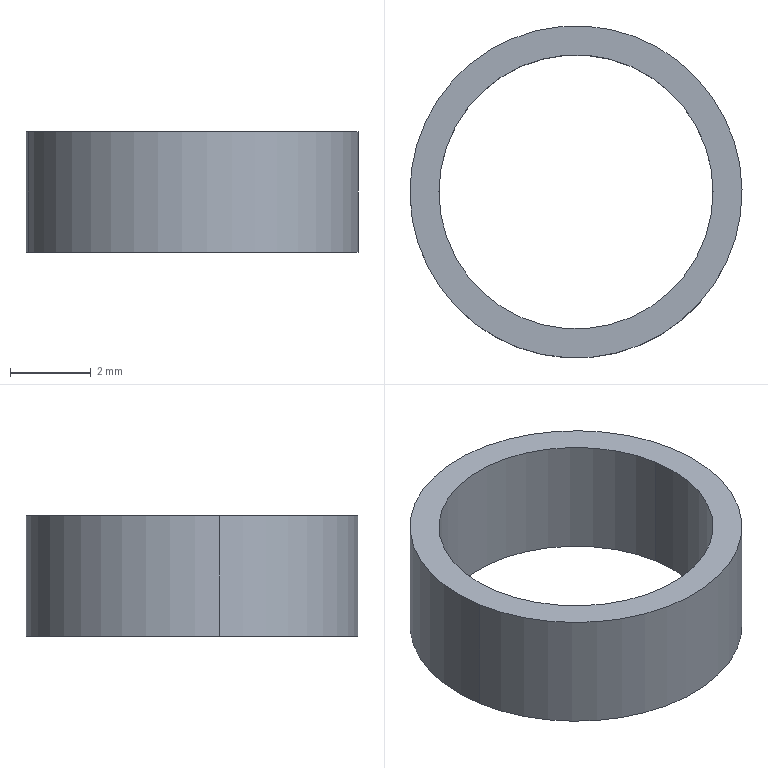Component | SolidWorks | Washer-1 | 1 solid | 6 faces | box 8.24 x 8.24 x 3 mm | volume 51 mm3 | cylinder 4 | plane 2 | commonest cylinder face diameters 6.8 x2 8.237 x2
build123d program:
from build123d import *

# Parameters (mm, degrees)
SKETCH2_R           = 4.118
SKETCH2_R_2         = 3.4
BOSS_EXTRUDE1_DEPTH = 3


with BuildPart() as part:
    # Sketch2 → Boss-Extrude1 (new body)
    with BuildSketch(Plane.XY.offset(7.373)):
        with Locations((105.719, -28.485)):
            Circle(SKETCH2_R)
        with Locations((105.719, -28.485)):
            Circle(SKETCH2_R_2, mode=Mode.SUBTRACT)
    extrude(amount=BOSS_EXTRUDE1_DEPTH)


solid = part.part

# Placed as in the assembly
solid = solid.moved(Location((-211.438, 0, 176.627), (0, 0, 0)))
STEP:
#1=COLOUR_RGB('',0.7922,0.8196,0.9333);
#2=FILL_AREA_STYLE_COLOUR('',#1);
#3=FILL_AREA_STYLE('',(#2));
#4=SURFACE_STYLE_FILL_AREA(#3);
#5=SURFACE_SIDE_STYLE('',(#4));
#6=SURFACE_STYLE_USAGE(.BOTH.,#5);
#7=PRESENTATION_STYLE_ASSIGNMENT((#6));
#8=CARTESIAN_POINT('',(-4.03,-1.099,7.244));
#9=VERTEX_POINT('',#8);
#10=CARTESIAN_POINT('',(-4.294,-1.144,7.244));
#11=VERTEX_POINT('',#10);
#12=CARTESIAN_POINT('',(-4.162,-1.121,7.244));
#13=DIRECTION('',(0.,0.,-1.));
#14=DIRECTION('',(-0.9863,-0.165,0.));
#15=AXIS2_PLACEMENT_3D('',#12,#13,#14);
#16=CIRCLE('',#15,0.1339);
#17=EDGE_CURVE('',#9,#11,#16,.T.);
#18=ORIENTED_EDGE('',*,*,#17,.T.);
#19=CARTESIAN_POINT('',(-4.294,-1.144,7.362));
#20=VERTEX_POINT('',#19);
#21=CARTESIAN_POINT('',(-4.294,-1.144,7.244));
#22=DIRECTION('',(-0.,-0.,1.));
#23=VECTOR('',#22,39.37);
#24=LINE('',#21,#23);
#25=EDGE_CURVE('',#11,#20,#24,.T.);
#26=ORIENTED_EDGE('',*,*,#25,.T.);
#27=CARTESIAN_POINT('',(-4.03,-1.099,7.362));
#28=VERTEX_POINT('',#27);
#29=CARTESIAN_POINT('',(-4.162,-1.121,7.362));
#30=DIRECTION('',(0.,0.,-1.));
#31=DIRECTION('',(-0.9863,-0.165,0.));
#32=AXIS2_PLACEMENT_3D('',#29,#30,#31);
#33=CIRCLE('',#32,0.1339);
#34=EDGE_CURVE('',#28,#20,#33,.T.);
#35=ORIENTED_EDGE('',*,*,#34,.F.);
#36=CARTESIAN_POINT('',(-4.03,-1.099,7.244));
#37=DIRECTION('',(-0.,-0.,1.));
#38=VECTOR('',#37,39.37);
#39=LINE('',#36,#38);
#40=EDGE_CURVE('',#9,#28,#39,.T.);
#41=ORIENTED_EDGE('',*,*,#40,.F.);
#42=EDGE_LOOP('',(#18,#26,#35,#41));
#43=FACE_OUTER_BOUND('',#42,.T.);
#44=CARTESIAN_POINT('',(-4.162,-1.121,7.244));
#45=DIRECTION('',(-0.,-0.,1.));
#46=DIRECTION('',(0.9863,0.165,0.));
#47=AXIS2_PLACEMENT_3D('',#44,#45,#46);
#48=CYLINDRICAL_SURFACE('',#47,0.1339);
#49=ADVANCED_FACE('',(#43),#48,.F.);
#50=CARTESIAN_POINT('',(-4.322,-1.148,7.244));
#51=VERTEX_POINT('',#50);
#52=CARTESIAN_POINT('',(-4.002,-1.095,7.244));
#53=VERTEX_POINT('',#52);
#54=CARTESIAN_POINT('',(-4.162,-1.121,7.244));
#55=DIRECTION('',(0.,0.,-1.));
#56=DIRECTION('',(-0.9863,-0.165,0.));
#57=AXIS2_PLACEMENT_3D('',#54,#55,#56);
#58=CIRCLE('',#57,0.1621);
#59=EDGE_CURVE('',#51,#53,#58,.T.);
#60=ORIENTED_EDGE('',*,*,#59,.F.);
#61=CARTESIAN_POINT('',(-4.322,-1.148,7.362));
#62=VERTEX_POINT('',#61);
#63=CARTESIAN_POINT('',(-4.322,-1.148,7.244));
#64=DIRECTION('',(-0.,-0.,1.));
#65=VECTOR('',#64,39.37);
#66=LINE('',#63,#65);
#67=EDGE_CURVE('',#51,#62,#66,.T.);
#68=ORIENTED_EDGE('',*,*,#67,.T.);
#69=CARTESIAN_POINT('',(-4.002,-1.095,7.362));
#70=VERTEX_POINT('',#69);
#71=CARTESIAN_POINT('',(-4.162,-1.121,7.362));
#72=DIRECTION('',(0.,0.,-1.));
#73=DIRECTION('',(-0.9863,-0.165,0.));
#74=AXIS2_PLACEMENT_3D('',#71,#72,#73);
#75=CIRCLE('',#74,0.1621);
#76=EDGE_CURVE('',#62,#70,#75,.T.);
#77=ORIENTED_EDGE('',*,*,#76,.T.);
#78=CARTESIAN_POINT('',(-4.002,-1.095,7.244));
#79=DIRECTION('',(-0.,-0.,1.));
#80=VECTOR('',#79,39.37);
#81=LINE('',#78,#80);
#82=EDGE_CURVE('',#53,#70,#81,.T.);
#83=ORIENTED_EDGE('',*,*,#82,.F.);
#84=EDGE_LOOP('',(#60,#68,#77,#83));
#85=FACE_OUTER_BOUND('',#84,.T.);
#86=CARTESIAN_POINT('',(-4.162,-1.121,7.244));
#87=DIRECTION('',(-0.,-0.,1.));
#88=DIRECTION('',(0.9863,0.165,0.));
#89=AXIS2_PLACEMENT_3D('',#86,#87,#88);
#90=CYLINDRICAL_SURFACE('',#89,0.1621);
#91=ADVANCED_FACE('',(#85),#90,.T.);
#92=CARTESIAN_POINT('',(-4.162,-1.121,7.244));
#93=DIRECTION('',(0.,0.,-1.));
#94=DIRECTION('',(-0.9863,-0.165,0.));
#95=AXIS2_PLACEMENT_3D('',#92,#93,#94);
#96=CIRCLE('',#95,0.1621);
#97=EDGE_CURVE('',#53,#51,#96,.T.);
#98=ORIENTED_EDGE('',*,*,#97,.T.);
#99=ORIENTED_EDGE('',*,*,#59,.T.);
#100=EDGE_LOOP('',(#98,#99));
#101=FACE_OUTER_BOUND('',#100,.T.);
#102=ORIENTED_EDGE('',*,*,#17,.F.);
#103=CARTESIAN_POINT('',(-4.162,-1.121,7.244));
#104=DIRECTION('',(0.,0.,-1.));
#105=DIRECTION('',(-0.9863,-0.165,0.));
#106=AXIS2_PLACEMENT_3D('',#103,#104,#105);
#107=CIRCLE('',#106,0.1339);
#108=EDGE_CURVE('',#11,#9,#107,.T.);
#109=ORIENTED_EDGE('',*,*,#108,.F.);
#110=EDGE_LOOP('',(#102,#109));
#111=FACE_BOUND('',#110,.T.);
#112=CARTESIAN_POINT('',(-4.162,-1.121,7.244));
#113=DIRECTION('',(0.,0.,-1.));
#114=DIRECTION('',(-0.9863,-0.165,-0.));
#115=AXIS2_PLACEMENT_3D('',#112,#113,#114);
#116=PLANE('',#115);
#117=ADVANCED_FACE('',(#101,#111),#116,.T.);
#118=CARTESIAN_POINT('',(-4.162,-1.121,7.362));
#119=DIRECTION('',(0.,0.,-1.));
#120=DIRECTION('',(-0.9863,-0.165,0.));
#121=AXIS2_PLACEMENT_3D('',#118,#119,#120);
#122=CIRCLE('',#121,0.1621);
#123=EDGE_CURVE('',#70,#62,#122,.T.);
#124=ORIENTED_EDGE('',*,*,#123,.F.);
#125=ORIENTED_EDGE('',*,*,#76,.F.);
#126=EDGE_LOOP('',(#124,#125));
#127=FACE_OUTER_BOUND('',#126,.T.);
#128=ORIENTED_EDGE('',*,*,#34,.T.);
#129=CARTESIAN_POINT('',(-4.162,-1.121,7.362));
#130=DIRECTION('',(0.,0.,-1.));
#131=DIRECTION('',(-0.9863,-0.165,0.));
#132=AXIS2_PLACEMENT_3D('',#129,#130,#131);
#133=CIRCLE('',#132,0.1339);
#134=EDGE_CURVE('',#20,#28,#133,.T.);
#135=ORIENTED_EDGE('',*,*,#134,.T.);
#136=EDGE_LOOP('',(#128,#135));
#137=FACE_BOUND('',#136,.T.);
#138=CARTESIAN_POINT('',(-4.162,-1.121,7.362));
#139=DIRECTION('',(0.,0.,-1.));
#140=DIRECTION('',(-0.9863,-0.165,-0.));
#141=AXIS2_PLACEMENT_3D('',#138,#139,#140);
#142=PLANE('',#141);
#143=ADVANCED_FACE('',(#127,#137),#142,.F.);
#144=ORIENTED_EDGE('',*,*,#67,.F.);
#145=ORIENTED_EDGE('',*,*,#97,.F.);
#146=ORIENTED_EDGE('',*,*,#82,.T.);
#147=ORIENTED_EDGE('',*,*,#123,.T.);
#148=EDGE_LOOP('',(#144,#145,#146,#147));
#149=FACE_OUTER_BOUND('',#148,.T.);
#150=CARTESIAN_POINT('',(-4.162,-1.121,7.244));
#151=DIRECTION('',(-0.,-0.,1.));
#152=DIRECTION('',(0.9863,0.165,0.));
#153=AXIS2_PLACEMENT_3D('',#150,#151,#152);
#154=CYLINDRICAL_SURFACE('',#153,0.1621);
#155=ADVANCED_FACE('',(#149),#154,.T.);
#156=ORIENTED_EDGE('',*,*,#25,.F.);
#157=ORIENTED_EDGE('',*,*,#108,.T.);
#158=ORIENTED_EDGE('',*,*,#40,.T.);
#159=ORIENTED_EDGE('',*,*,#134,.F.);
#160=EDGE_LOOP('',(#156,#157,#158,#159));
#161=FACE_OUTER_BOUND('',#160,.T.);
#162=CARTESIAN_POINT('',(-4.162,-1.121,7.244));
#163=DIRECTION('',(-0.,-0.,1.));
#164=DIRECTION('',(0.9863,0.165,0.));
#165=AXIS2_PLACEMENT_3D('',#162,#163,#164);
#166=CYLINDRICAL_SURFACE('',#165,0.1339);
#167=ADVANCED_FACE('',(#161),#166,.F.);
#168=CLOSED_SHELL('',(#49,#91,#117,#143,#155,#167));
#169=MANIFOLD_SOLID_BREP('',#168);
#170=STYLED_ITEM('',(#7),#169);
#171=(LENGTH_UNIT()NAMED_UNIT(*)SI_UNIT($,.METRE.));
#172=LENGTH_MEASURE_WITH_UNIT(LENGTH_MEASURE(0.0254),#171);
#173=DIMENSIONAL_EXPONENTS(1.,0.,0.,0.,0.,0.,0.);
#174=(CONVERSION_BASED_UNIT('',#172)LENGTH_UNIT()NAMED_UNIT(#173));
#175=UNCERTAINTY_MEASURE_WITH_UNIT(LENGTH_MEASURE(0.00001),#174,'','');
#176=(NAMED_UNIT(*)PLANE_ANGLE_UNIT()SI_UNIT($,.RADIAN.));
#177=(NAMED_UNIT(*)SI_UNIT($,.STERADIAN.)SOLID_ANGLE_UNIT());
#178=(GEOMETRIC_REPRESENTATION_CONTEXT(3)GLOBAL_UNCERTAINTY_ASSIGNED_CONTEXT((#175))GLOBAL_UNIT_ASSIGNED_CONTEXT((#174,#176,#177))REPRESENTATION_CONTEXT('',''));
#179=MECHANICAL_DESIGN_GEOMETRIC_PRESENTATION_REPRESENTATION('',(#170),#178);
#180=PRESENTATION_LAYER_ASSIGNMENT('','',(#170));
#181=CARTESIAN_POINT('',(0.,0.,0.));
#182=DIRECTION('',(0.,0.,1.));
#183=DIRECTION('',(1.,0.,0.));
#184=AXIS2_PLACEMENT_3D('',#181,#182,#183);
#185=(LENGTH_UNIT()NAMED_UNIT(*)SI_UNIT($,.METRE.));
#186=LENGTH_MEASURE_WITH_UNIT(LENGTH_MEASURE(0.0254),#185);
#187=DIMENSIONAL_EXPONENTS(1.,0.,0.,0.,0.,0.,0.);
#188=(CONVERSION_BASED_UNIT('',#186)LENGTH_UNIT()NAMED_UNIT(#187));
#189=UNCERTAINTY_MEASURE_WITH_UNIT(LENGTH_MEASURE(0.00001),#188,'','');
#190=(NAMED_UNIT(*)PLANE_ANGLE_UNIT()SI_UNIT($,.RADIAN.));
#191=(NAMED_UNIT(*)SI_UNIT($,.STERADIAN.)SOLID_ANGLE_UNIT());
#192=(GEOMETRIC_REPRESENTATION_CONTEXT(3)GLOBAL_UNCERTAINTY_ASSIGNED_CONTEXT((#189))GLOBAL_UNIT_ASSIGNED_CONTEXT((#188,#190,#191))REPRESENTATION_CONTEXT('',''));
#193=ADVANCED_BREP_SHAPE_REPRESENTATION('',(#169,#184),#192);